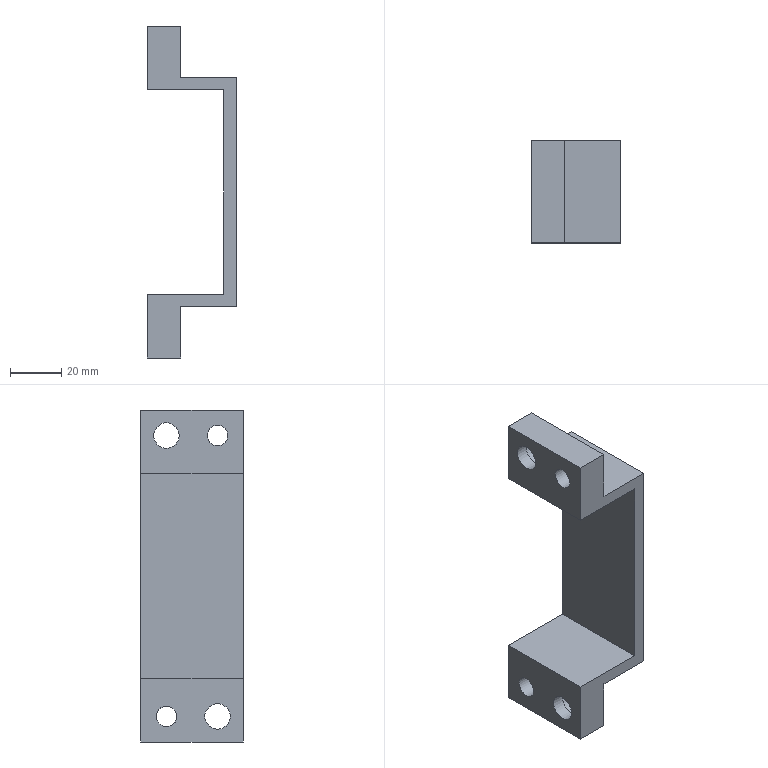Component | NX | MOVABLE_BASE | 1 solid | 22 faces | volume 46584 mm3 | plane 16 | cylinder 6 | commonest cylinder face diameters 10 x2 13 x2 8 x2